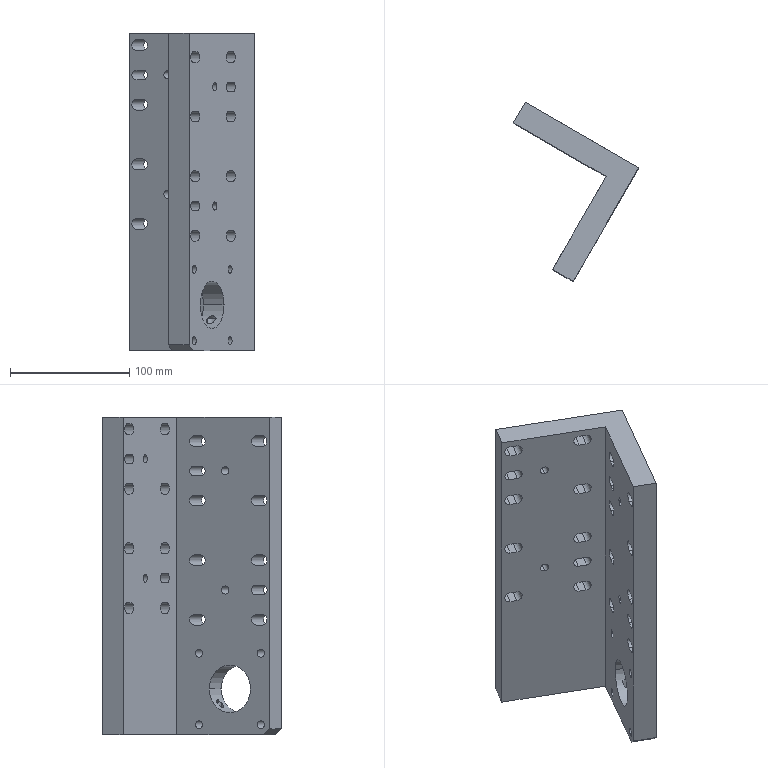Component | SolidWorks | KLHFH004LocatingSeatConnectingFixingPlate-SymmetricPart-1 | 1 solid | 130 faces | volume 979721 mm3 | cylinder 70 | plane 49 | cone 11 | commonest cylinder face diameters 9 x32 6.8 x16 8 x12 8.5 x8 40 x2 | material Plain Carbon Steel